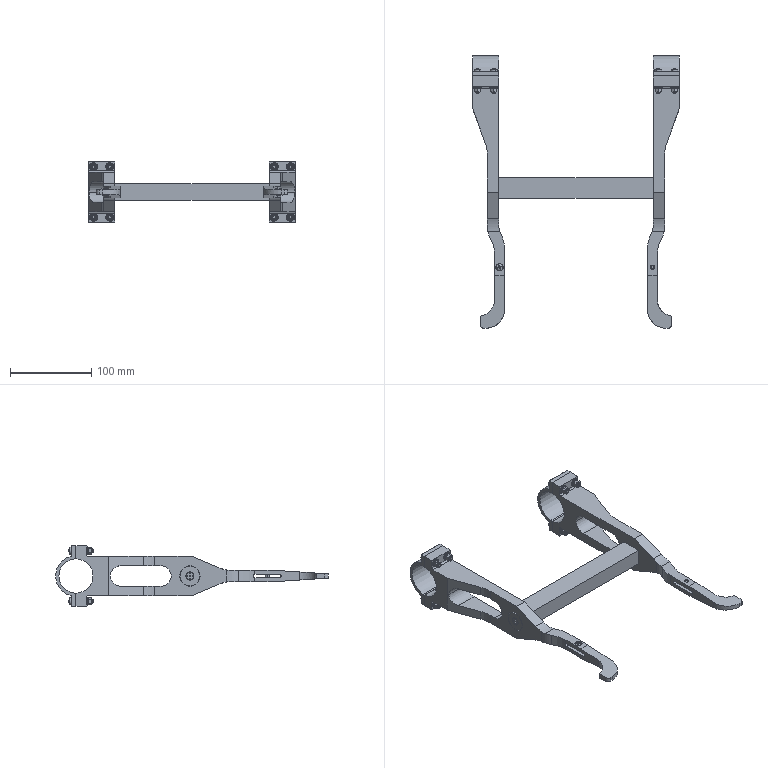Assembly | SolidWorks | mm | 43 component files | 43 solids | 1842 faces | box 254 x 335 x 74 mm | volume 383562 mm3 | cone 1140 | plane 386 | cylinder 272 | torus 24 | sphere 20 | commonest cylinder face diameters 5 x72 4.33 x24 10 x20 8.5 x20 5.8 x16 5.2 x16 7.5 x16 5.3 x16
Bill of materials:
AxleSupport | 2 |  | Long, flat, tapering arm. The wide end is a fork with two block-shaped bosses and a concave arc cut between them. The narrow end bends into a curved, hook-like tip.
Beam | 1 |  | Straight bar with a rectangular cross-section. Each end has a smaller, stepped-down rectangular stub, and one stub has a small round hole in its end face.
Cover | 2 | 6061 Alloy | Saddle-shaped strap: a half-cylinder of constant thickness with a flat flange on each side, and two round holes through each flange.
GB 93-87-5 | 8 | AISI 321 Annealed Stainless Steel (SS) | Split ring with a rectangular cross-section and a single radial gap. It looks like a split washer.
GB_T6170-2000Type1HexNutGradeAAndBM5 | 8 | AISI 321 Annealed Stainless Steel (SS) | Hexagonal prism with a central round through-bore and chamfered corners. It looks like a hex nut.
GB_T818-2000PhillipsPanHeadScrewM5_10 | 2 |  | Headed pin with a plain cylindrical shank and a chamfered tip. The shank necks down above a round head, and the head's underside is domed with a slot.
GB_T818-2000PhillipsPanHeadScrewM5_25 | 8 |  | Screw with a threaded shank, a short undercut neck, and a cylindrical head with a rounded top and a recessed drive.
GB_T819.1-2000PhillipsCountersunkHeadScrewM5_20 | 2 |  | Countersunk, flat-headed fastener-like part. It has a conical head, a short filleted neck and a plain cylindrical shank with a chamfered end.
GB_T97.2-1985FlatWasherChamferedTypeA5_1 | 8 | AISI 321 Annealed Stainless Steel (SS) | Thin flat ring with a central round hole. It looks like a plain washer, with a chamfer on one outer edge.
Pillar-BeamConnectionGasket | 2 |  | Thick cylindrical disc with a small central through-hole. It could be a spacer, a thick washer or a wheel blank.
Mates:
1. coincident | Beam-1 face at (-242.428, 20.796, 291.382) dir (0, 0, 1) | AxleSupport-1 face at (-265.428, 34.796, 291.382) dir (0, 0, -1)
2. coincident | Beam-1 face at (-233.428, 50.643, 284.382) dir (-1, 0, 0) | AxleSupport-1 face at (-233.428, 167.796, 321.382) dir (1, 0, 0)
3. coincident | Cover-1 face at (-233.428, 167.796, 305.382) dir (0, -1, 0) | AxleSupport-1 face at (-233.428, 167.796, 321.382) dir (0, 1, 0)
4. concentric | Cover-1 face at (-239.428, 167.796, 315.382) dir (0, 1, 0) r 2.9 | AxleSupport-1 face at (-239.428, -142.205, 315.382) dir (0, 1, 0) r 2.5
5. concentric | Cover-1 face at (-259.428, 167.796, 253.382) dir (0, 1, 0) r 2.9 | AxleSupport-1 face at (-259.428, -142.205, 253.382) dir (0, 1, 0) r 2.5
6. coincident | AxleSupport-1 face at (-242.428, 27.796, 284.382) dir (-1, 0, 0) | Pillar-BeamConnectionGasket-1 face at (-242.428, 27.796, 284.382) dir (1, 0, 0)
7. concentric | Pillar-BeamConnectionGasket-1 face at (-242.428, 27.796, 284.382) dir (-1, 0, 0) r 2.5 | Beam-1 face at (-242.428, 27.796, 284.382) dir (-1, 0, 0) r 2.5
8. coincident | Beam-1 face at (-242.428, 20.796, 277.382) dir (0, -1, 0) | AxleSupport-1 face at (-265.428, 20.796, 291.382) dir (0, 1, 0)
9. concentric | Beam-1 face at (-242.428, 27.796, 284.382) dir (-1, 0, 0) r 2.5 | GB_T819.1-2000PhillipsCountersunkHeadScrewM5_20-1 face at (-247.293, 27.796, 284.382) dir (-1, 0, 0) r 2.5
10. coincident | Pillar-BeamConnectionGasket-1 face at (-244.928, 27.796, 284.382) dir (1, 0, 0) r 785.398 | GB_T819.1-2000PhillipsCountersunkHeadScrewM5_20-1 face at (-244.974, 27.796, 284.382) dir (1, 0, 0) r 785.398
11. concentric | Beam-1 face at (-34.428, 27.796, 284.382) dir (1, 0, 0) r 2.5 | GB_T819.1-2000PhillipsCountersunkHeadScrewM5_20-2 face at (-29.563, 27.796, 284.382) dir (1, 0, 0) r 2.5
12. coincident | Pillar-BeamConnectionGasket-2 face at (-31.928, 27.796, 284.382) dir (-1, 0, 0) r 785.398 | GB_T819.1-2000PhillipsCountersunkHeadScrewM5_20-2 face at (-31.883, 27.796, 284.382) dir (-1, 0, 0) r 785.398
13. concentric | AxleSupport-2 face at (-44.428, -67.204, 277.382) dir (0, 0, -1) r 2.5 | GB_T818-2000PhillipsPanHeadScrewM5_10-1 face at (-44.428, -67.204, 275.951) dir (0, 0, -1) r 2.5
14. coincident | AxleSupport-2 face at (-44.428, -67.204, 280.982) dir (0, 0, -1) | GB_T818-2000PhillipsPanHeadScrewM5_10-1 face at (-44.428, -64.354, 280.982) dir (0, 0, 1)
15. concentric | AxleSupport-1 face at (-232.428, -67.204, 291.382) dir (0, 0, 1) r 2.5 | GB_T818-2000PhillipsPanHeadScrewM5_10-2 face at (-232.428, -67.204, 292.814) dir (0, 0, 1) r 2.5
16. coincident | AxleSupport-1 face at (-232.428, -67.204, 287.782) dir (0, 0, 1) | GB_T818-2000PhillipsPanHeadScrewM5_10-2 face at (-233.52, -64.571, 287.782) dir (0, 0, -1)
17. concentric | Cover-1 face at (-259.428, 167.796, 315.382) dir (0, 1, 0) r 2.9 | GB_T818-2000PhillipsPanHeadScrewM5_25-1 face at (-259.428, 177.828, 315.382) dir (0, 1, 0) r 2.165
18. coincident | Cover-1 face at (-233.428, 172.796, 321.382) dir (0, 1, 0) | GB_T818-2000PhillipsPanHeadScrewM5_25-1 face at (-256.888, 172.796, 314.09) dir (0, -1, 0)
19. coincident | AxleSupport-1 face at (-265.428, 154.796, 284.382) dir (0, -1, 0) | GB_T97.2-1985FlatWasherChamferedTypeA5_1-1 face at (-257.21, 154.796, 316.832) dir (0, 1, 0)
20. concentric | GB_T818-2000PhillipsPanHeadScrewM5_25-1 face at (-259.428, 147.192, 315.382) dir (0, -1, 0) r 1051.888 | GB_T97.2-1985FlatWasherChamferedTypeA5_1-1 face at (-259.428, 163.441, 315.382) dir (0, 1, 0) r 2.65
21. concentric | GB 93-87-5-1 face at (-259.428, 153.796, 315.382) dir (0, -1, 0) r 2.6 | GB_T818-2000PhillipsPanHeadScrewM5_25-1 face at (-259.428, 147.192, 315.382) dir (0, -1, 0) r 1051.888
22. coincident | GB 93-87-5-1 face at (-259.428, 153.796, 315.382) dir (0, 1, 0) | GB_T97.2-1985FlatWasherChamferedTypeA5_1-1 face at (-257.21, 153.796, 316.832) dir (0, -1, 0)
23. coincident | GB 93-87-5-1 face at (-259.428, 152.796, 315.382) dir (0, -1, 0) | GB_T6170-2000Type1HexNutGradeAAndBM5-1 face at (-255.613, 152.796, 313.2) dir (0, 1, 0)
24. concentric | GB_T6170-2000Type1HexNutGradeAAndBM5-1 face at (-259.428, 152.796, 315.382) dir (0, -1, 0) r 2.5 | GB_T818-2000PhillipsPanHeadScrewM5_25-1 face at (-259.428, 147.192, 315.382) dir (0, -1, 0) r 1051.888